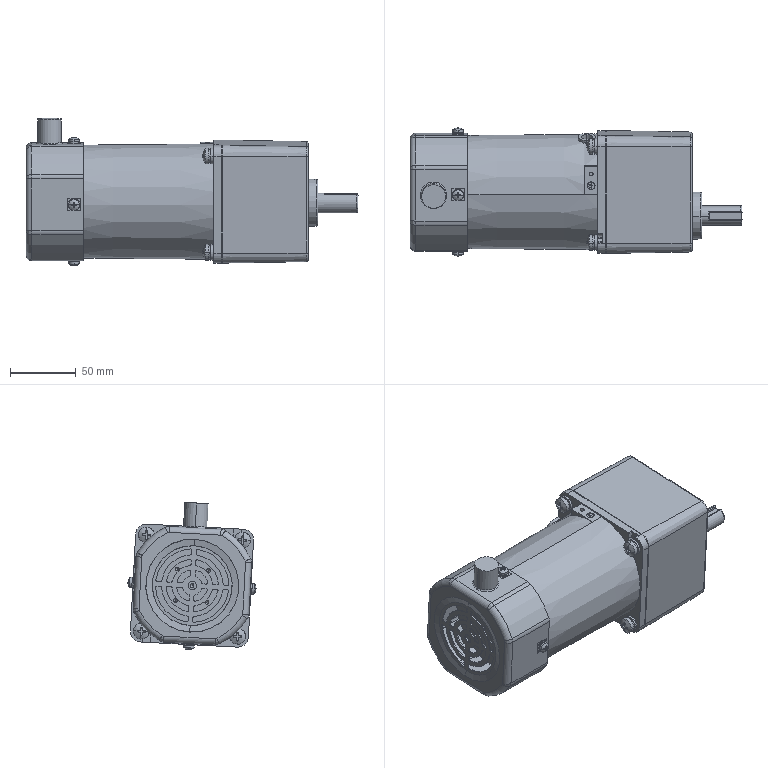Component | SolidWorks | StepperMotor-2 | 28 solids | 842 faces | volume 1250838 mm3 | cylinder 385 | plane 314 | cone 53 | torus 48 | sphere 24 | spline 18 | commonest cylinder face diameters 2 x53 0.6 x32 12 x22 4.4 x16 6.6 x16 4 x16 9 x16 6.68 x13